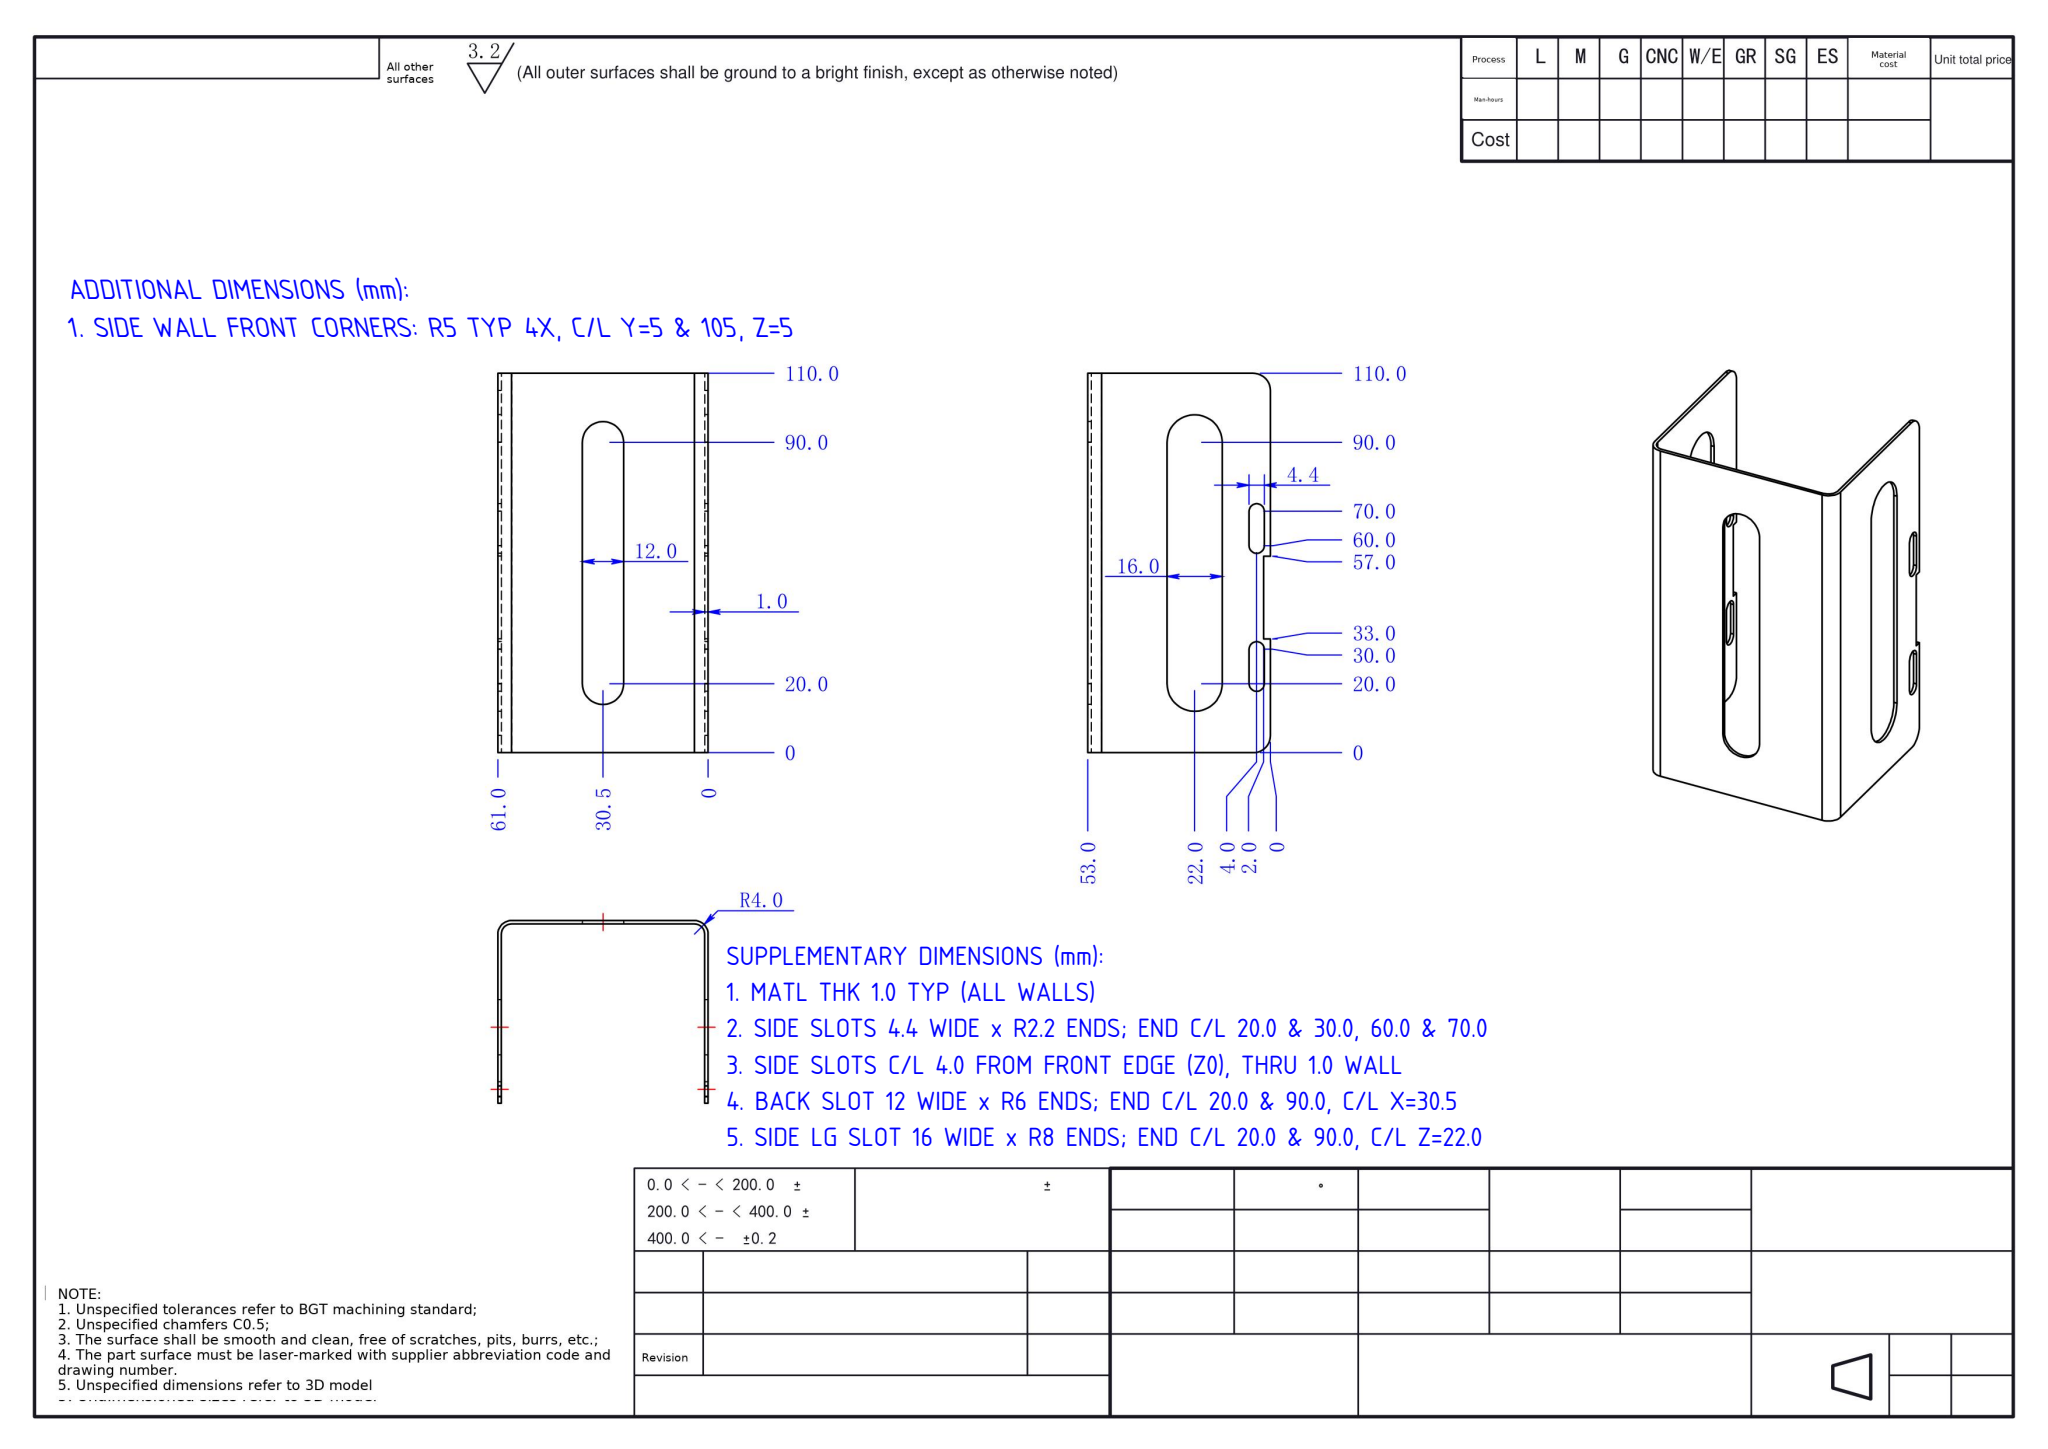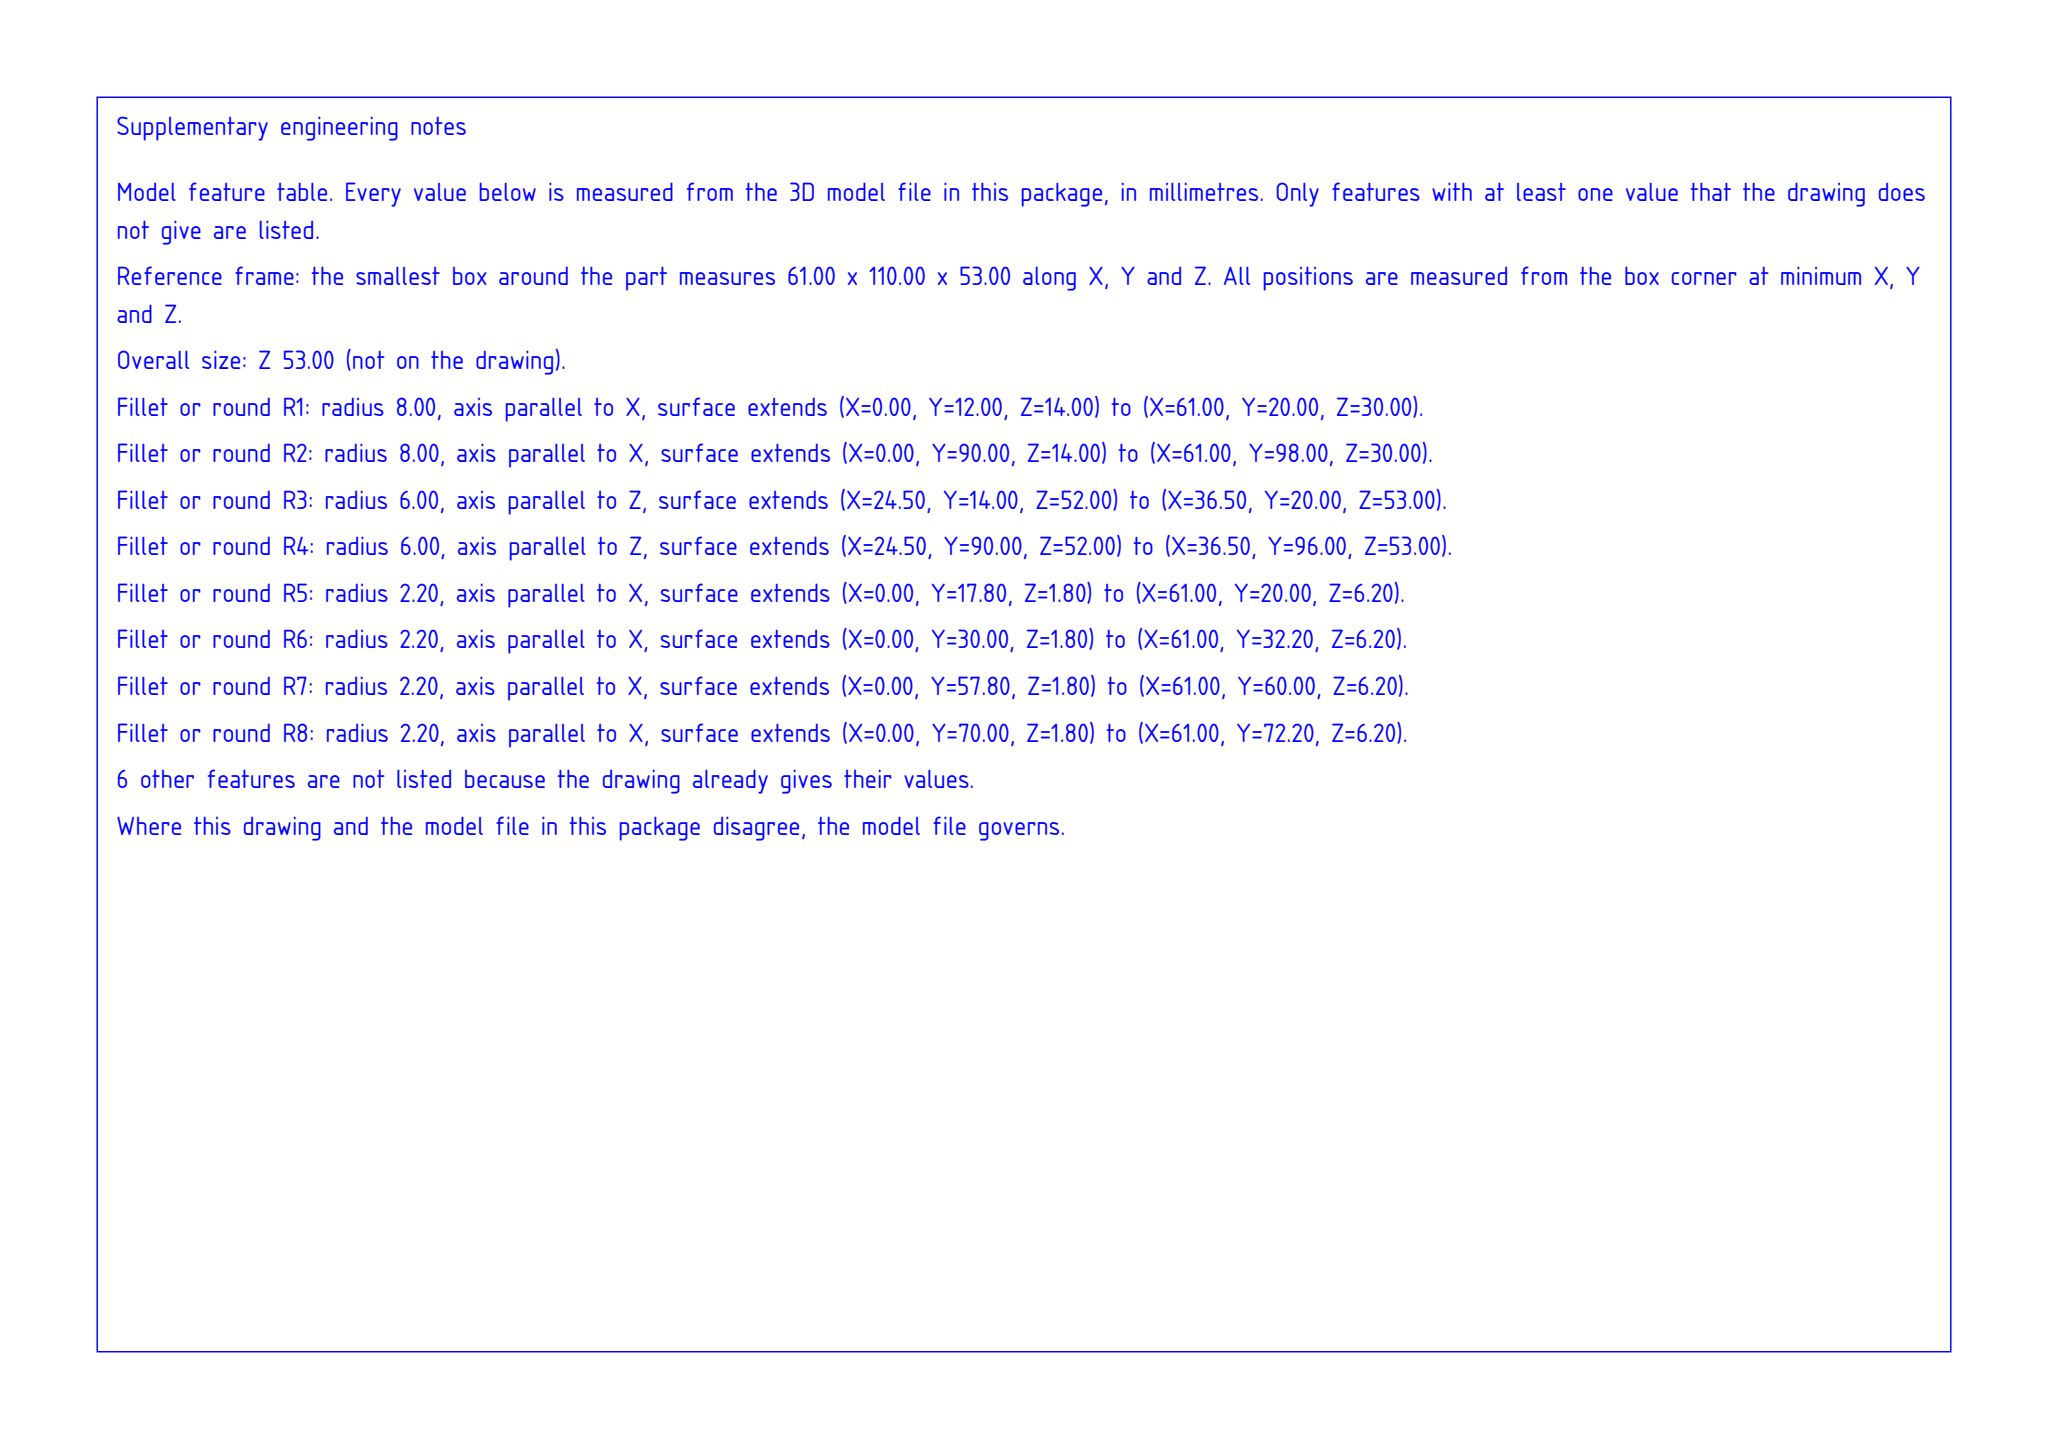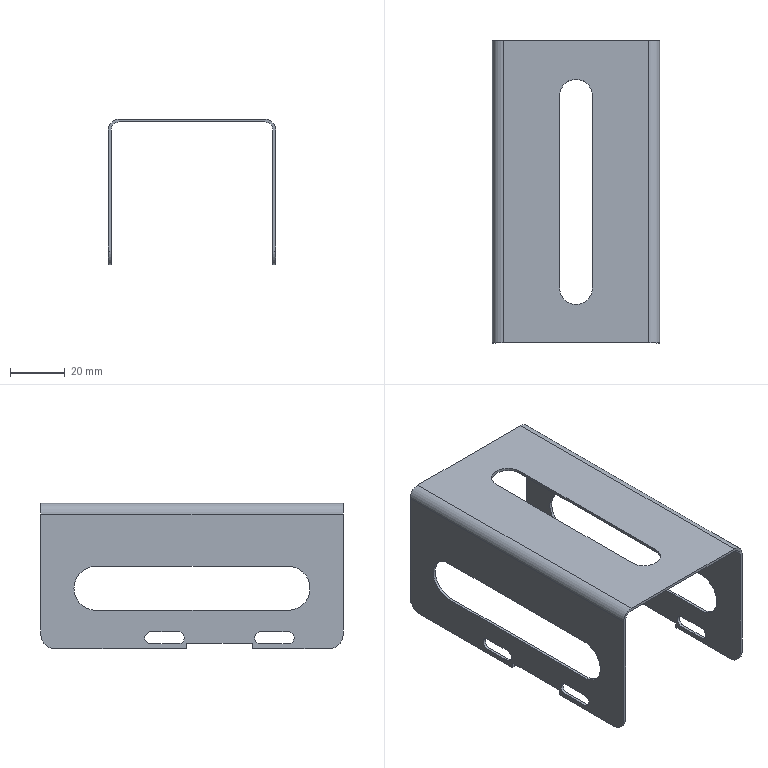Part | SolidWorks | mm | 1 solid | 60 faces | box 61 x 110 x 53 mm | volume 13870 mm3 | plane 32 | cylinder 28 | commonest cylinder face diameters 4.4 x12 16 x6 10 x4 8 x2 6 x2 12 x2
build123d program:
from build123d import *

# Parameters (mm, degrees)
SKETCH1_W           = 61
SKETCH1_H           = 110
BOSS_EXTRUDE1_DEPTH = 53
FILLET1_R           = 4
FILLET2_R           = 5
SHELL1_T            = -1
CUT_EXTRUDE2_DEPTH  = 2
CUT_EXTRUDE3_DEPTH  = 98.75
CUT_EXTRUDE4_DEPTH  = 98.75
SKETCH6_W           = 2
SKETCH6_H           = 24
CUT_EXTRUDE5_DEPTH  = 98.75


with BuildPart() as part:
    # Sketch1 → Boss-Extrude1 (new body)
    with BuildSketch(Plane.XY):
        Rectangle(SKETCH1_W, SKETCH1_H)
    extrude(amount=BOSS_EXTRUDE1_DEPTH)

    # Fillet1
    fillet1_edges = [part.edges().sort_by_distance(p)[0] for p in [
        (-30.5, 0, 53),
        (30.5, 0, 53),
    ]]
    fillet(fillet1_edges, radius=FILLET1_R)

    # Fillet2
    fillet2_edges = [part.edges().sort_by_distance(p)[0] for p in [
        (0, -55, 0),
        (0, 55, 0),
    ]]
    fillet(fillet2_edges, radius=FILLET2_R)

    # Shell1
    shell1_openings = [part.faces().sort_by_distance(p)[0] for p in [
        (0, -53.536, 1.464),
        (0, 53.536, 1.464),
        (0, 0, 0),
        (0, -55, 28.946),
        (0, 55, 28.946),
    ]]
    offset(amount=SHELL1_T, openings=shell1_openings, kind=Kind.INTERSECTION)

    # Sketch3 → Cut-Extrude2 (cut)
    with BuildSketch(Plane.XY.offset(53)):
        with BuildLine():
            Line((6, 35), (6, -35))
            ThreePointArc((6, -35), (0, -41), (-6, -35))
            Line((-6, -35), (-6, 35))
            ThreePointArc((-6, 35), (0, 41), (6, 35))
        make_face()
    extrude(amount=-CUT_EXTRUDE2_DEPTH, mode=Mode.SUBTRACT)

    # Sketch4 → Cut-Extrude3 (cut, through all)
    with BuildSketch(Plane(origin=(30.5, 0, 0), x_dir=(0, 0, -1), z_dir=(1, 0, 0))):
        with BuildLine():
            Line((-1.8, 15), (-1.8, 5))
            ThreePointArc((-1.8, 5), (-4, 2.8), (-6.2, 5))
            Line((-6.2, 5), (-6.2, 15))
            ThreePointArc((-6.2, 15), (-4, 17.2), (-1.8, 15))
        make_face()
        with BuildLine():
            Line((-1.8, -35), (-1.8, -25))
            ThreePointArc((-1.8, -25), (-4, -22.8), (-6.2, -25))
            Line((-6.2, -25), (-6.2, -35))
            ThreePointArc((-6.2, -35), (-4, -37.2), (-1.8, -35))
        make_face()
    extrude(amount=-CUT_EXTRUDE3_DEPTH, mode=Mode.SUBTRACT)

    # Sketch5 → Cut-Extrude4 (cut, through all)
    with BuildSketch(Plane(origin=(30.5, 0, 0), x_dir=(0, 0, -1), z_dir=(1, 0, 0))):
        with BuildLine():
            Line((-14, 35), (-14, -35))
            ThreePointArc((-14, -35), (-22, -43), (-30, -35))
            Line((-30, -35), (-30, 35))
            ThreePointArc((-30, 35), (-22, 43), (-14, 35))
        make_face()
    extrude(amount=-CUT_EXTRUDE4_DEPTH, mode=Mode.SUBTRACT)

    # Sketch6 → Cut-Extrude5 (cut, through all)
    with BuildSketch(Plane(origin=(30.5, 0, 0), x_dir=(0, 0, -1), z_dir=(1, 0, 0))):
        with Locations((-1, -10)):
            Rectangle(SKETCH6_W, SKETCH6_H)
    extrude(amount=-CUT_EXTRUDE5_DEPTH, mode=Mode.SUBTRACT)


solid = part.part